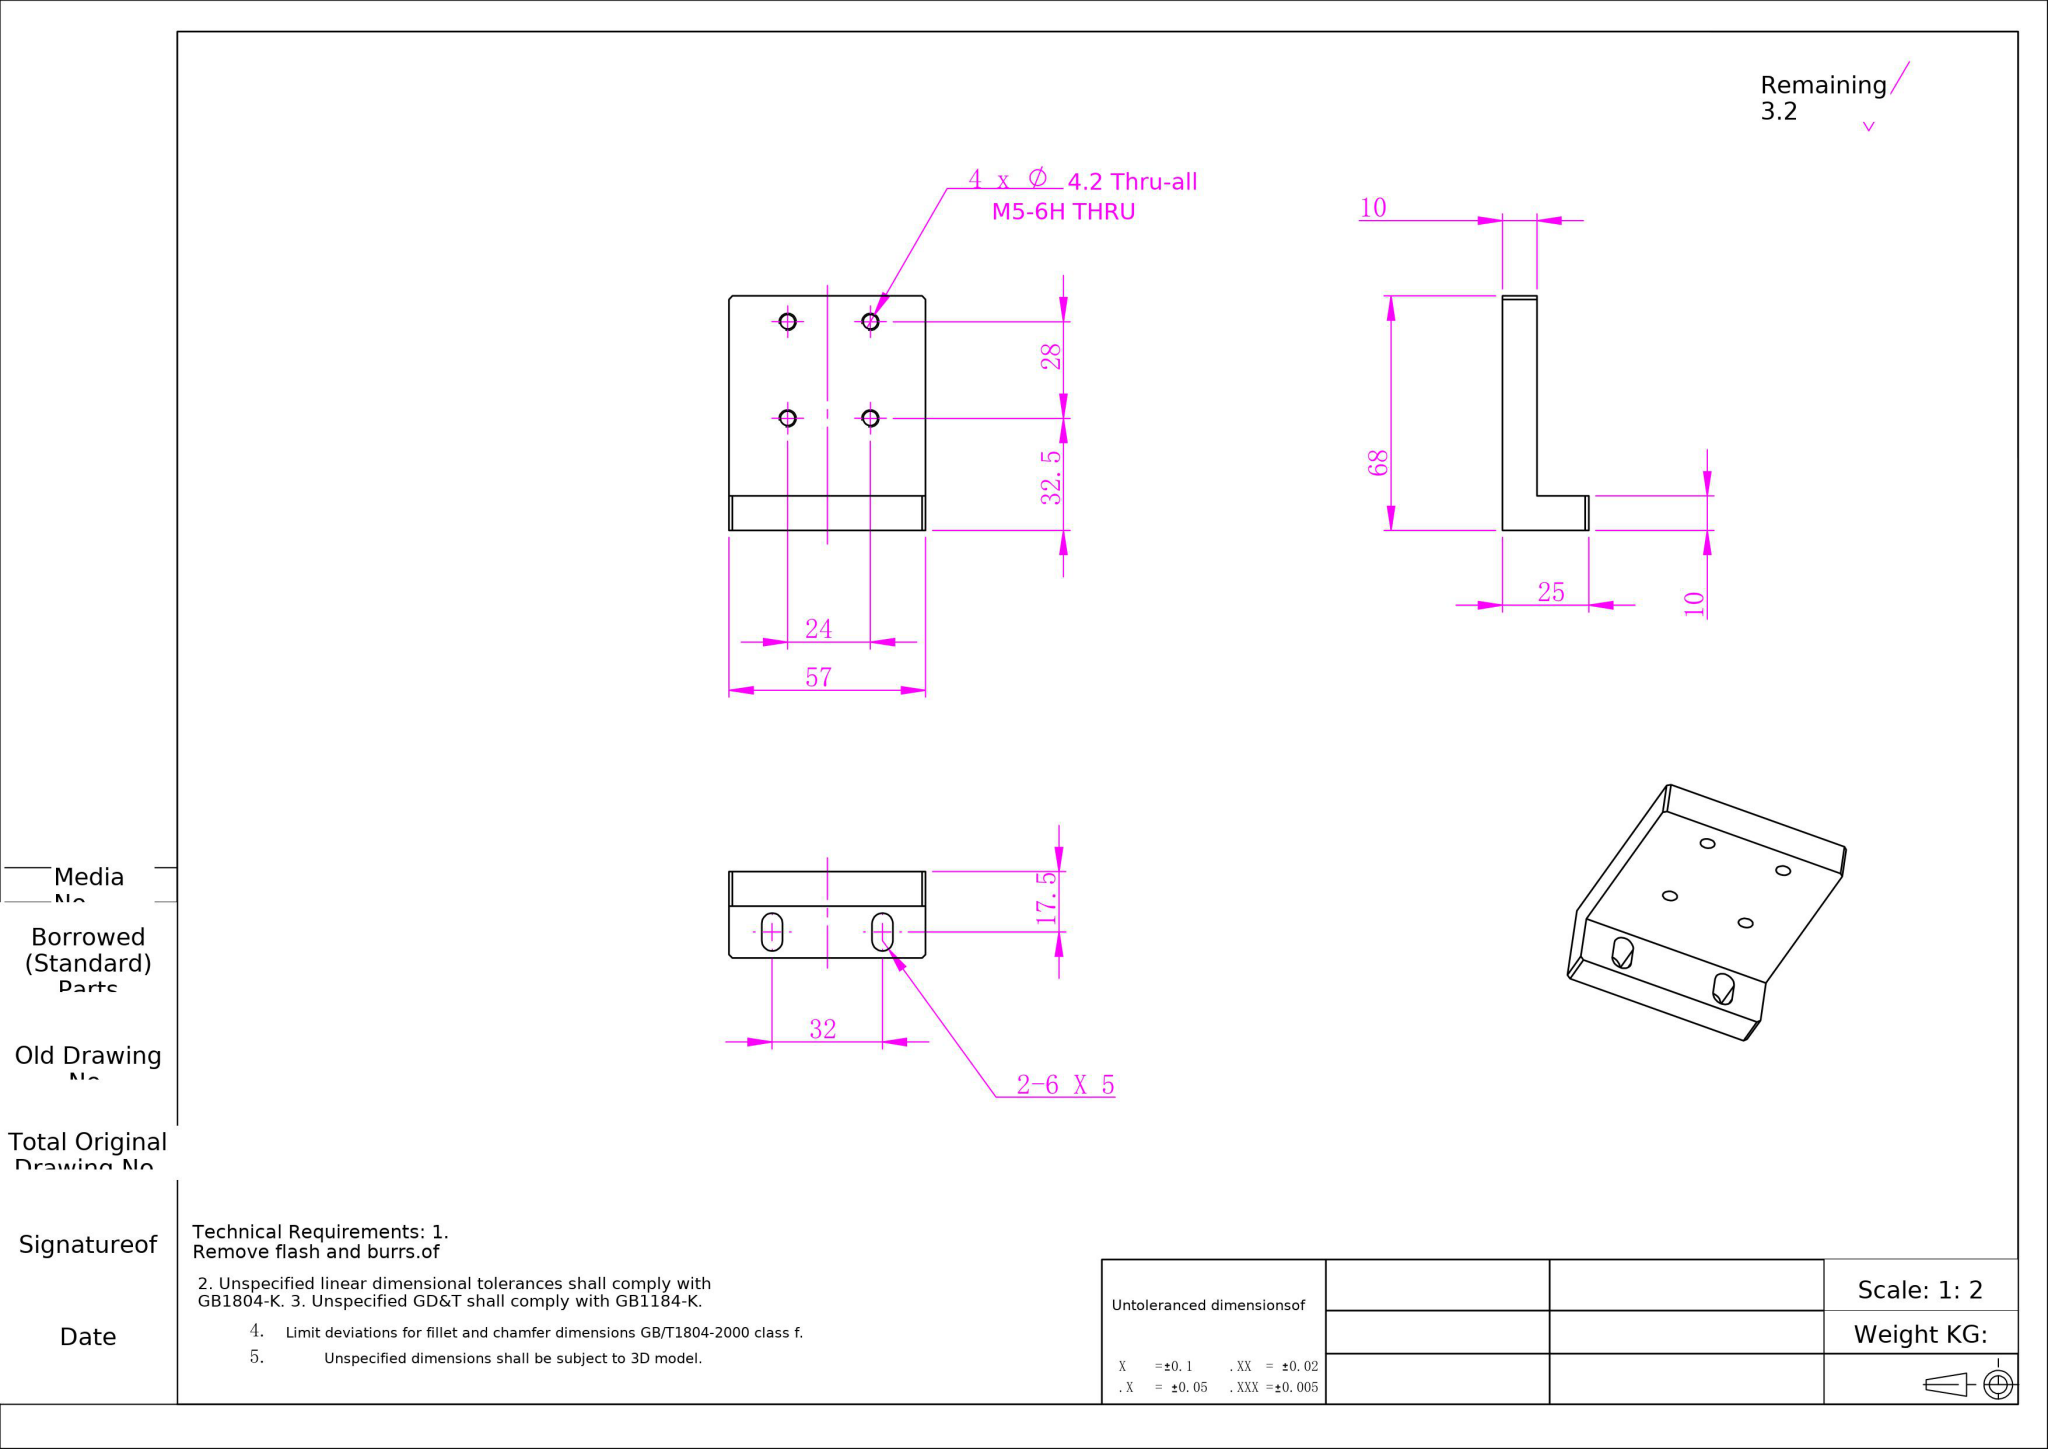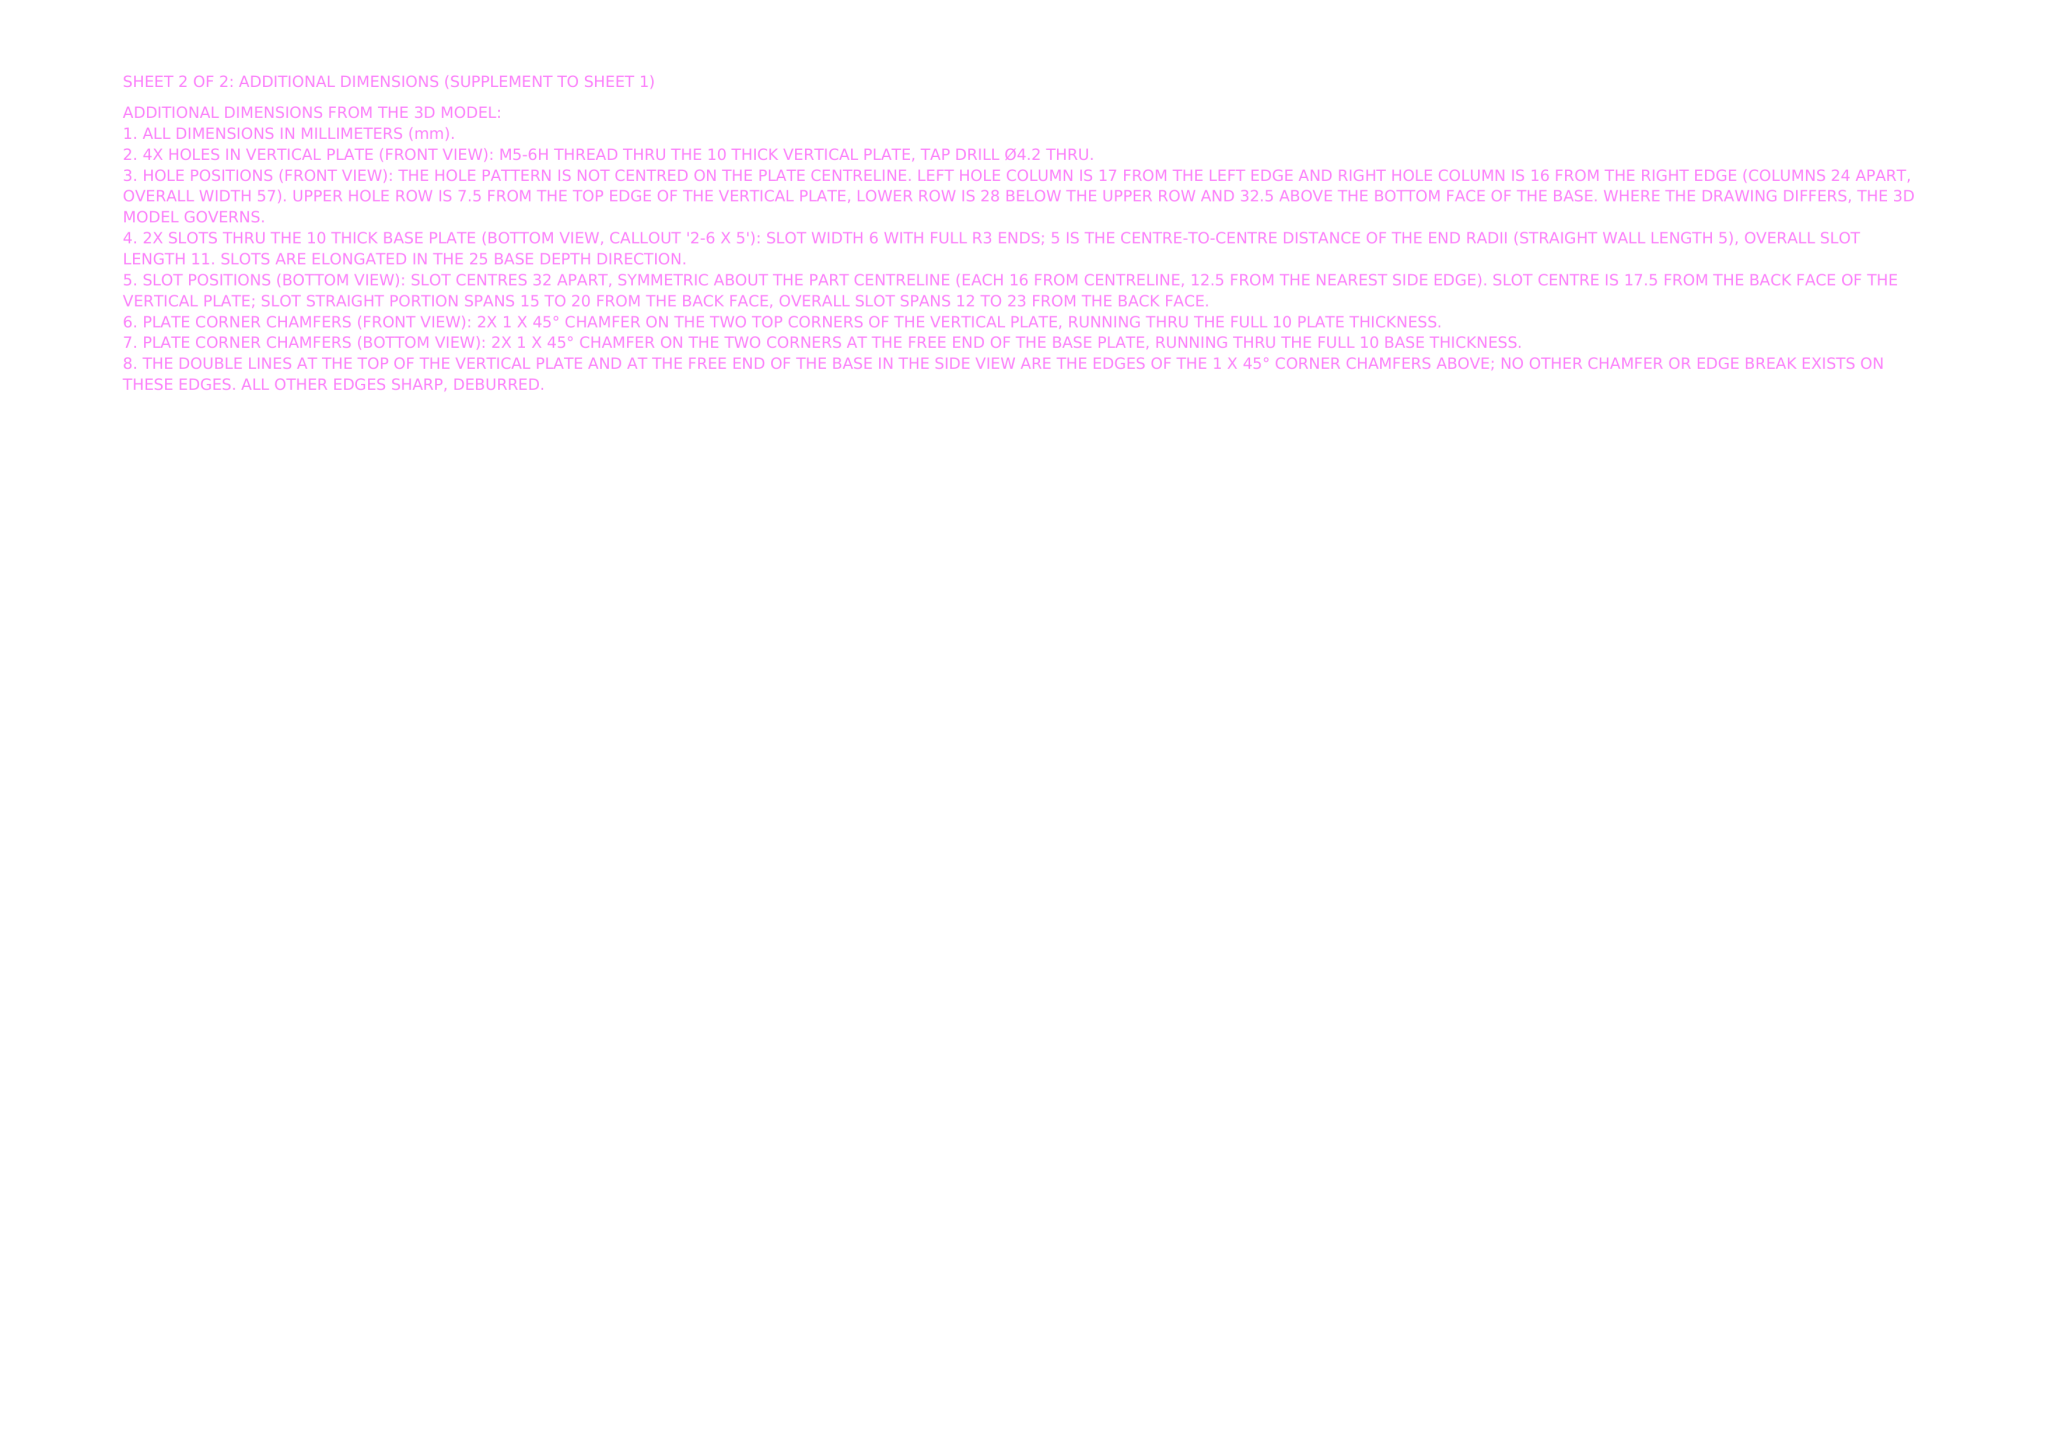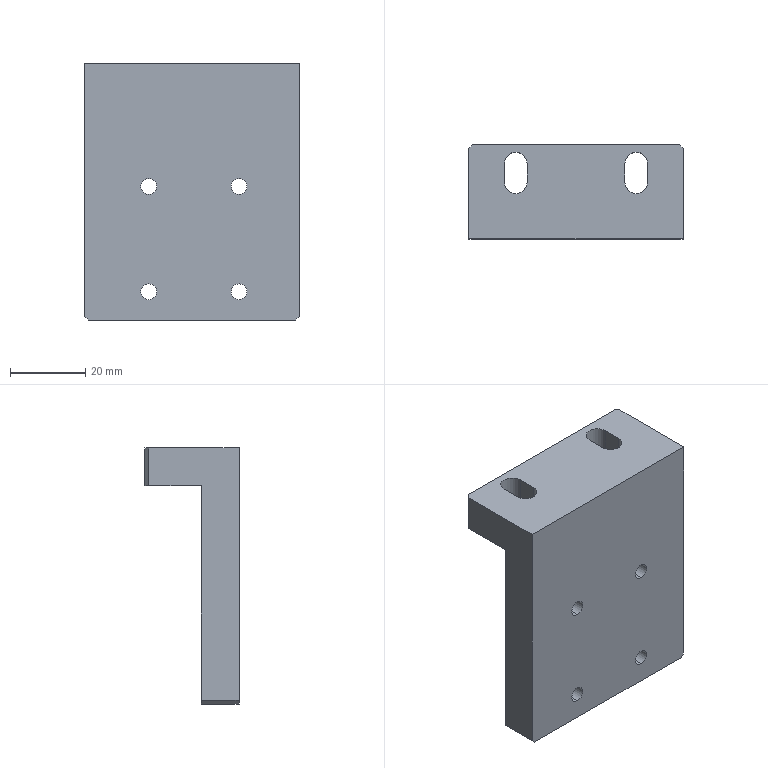Part | NX | mm | 1 solid | 28 faces | box 57 x 25 x 68 mm | volume 45570 mm3 | plane 16 | cylinder 12 | commonest cylinder face diameters 4.2 x8 6 x4